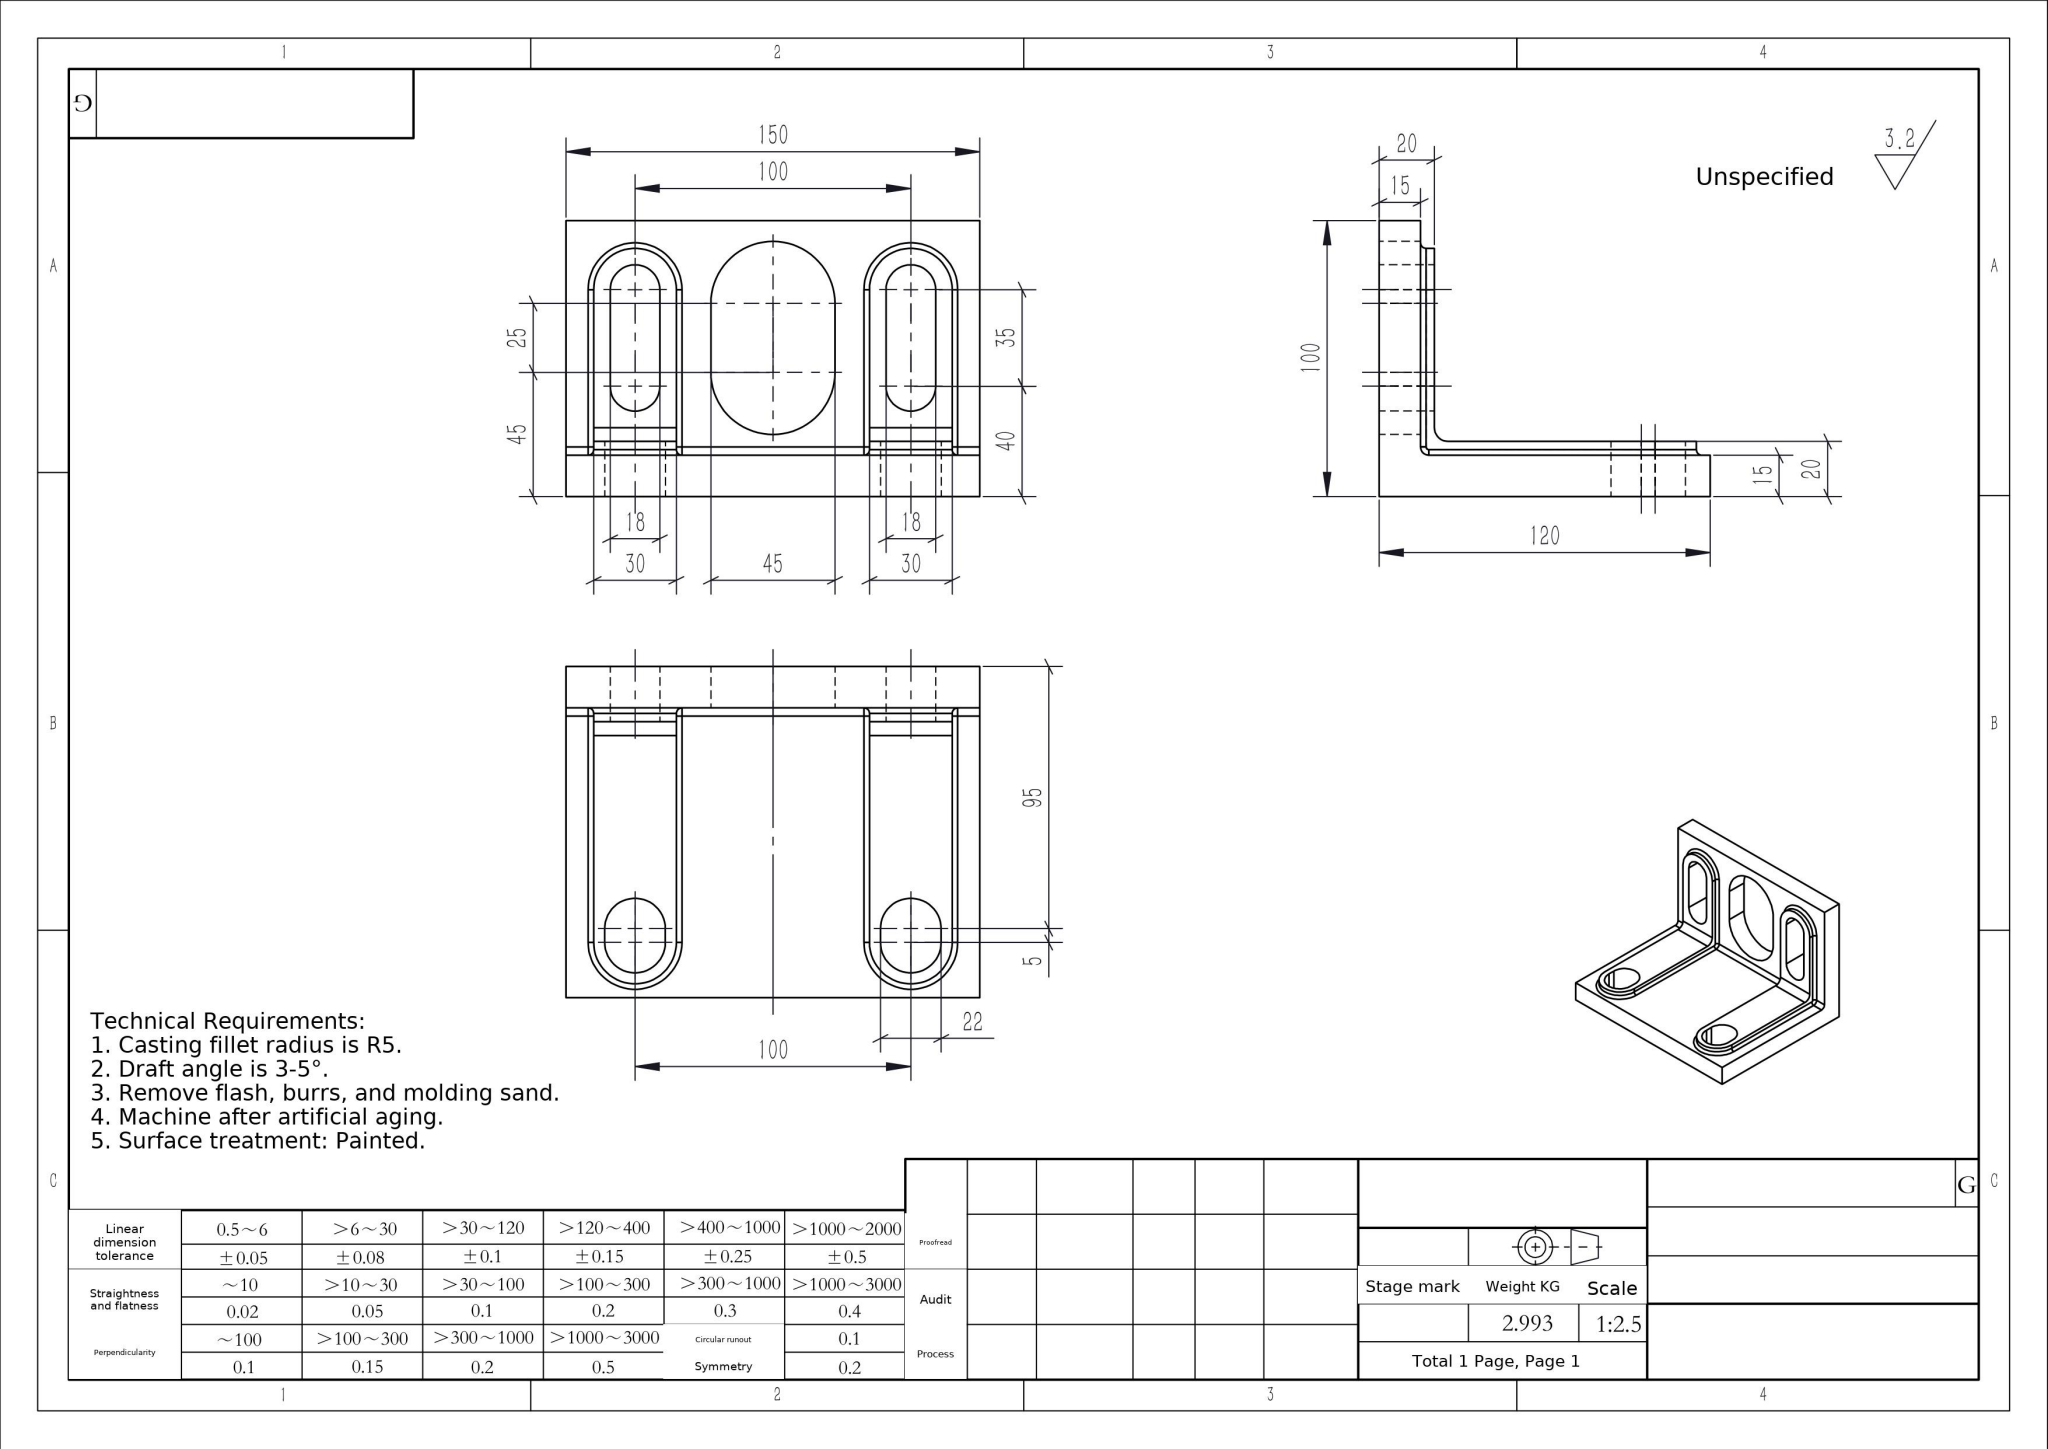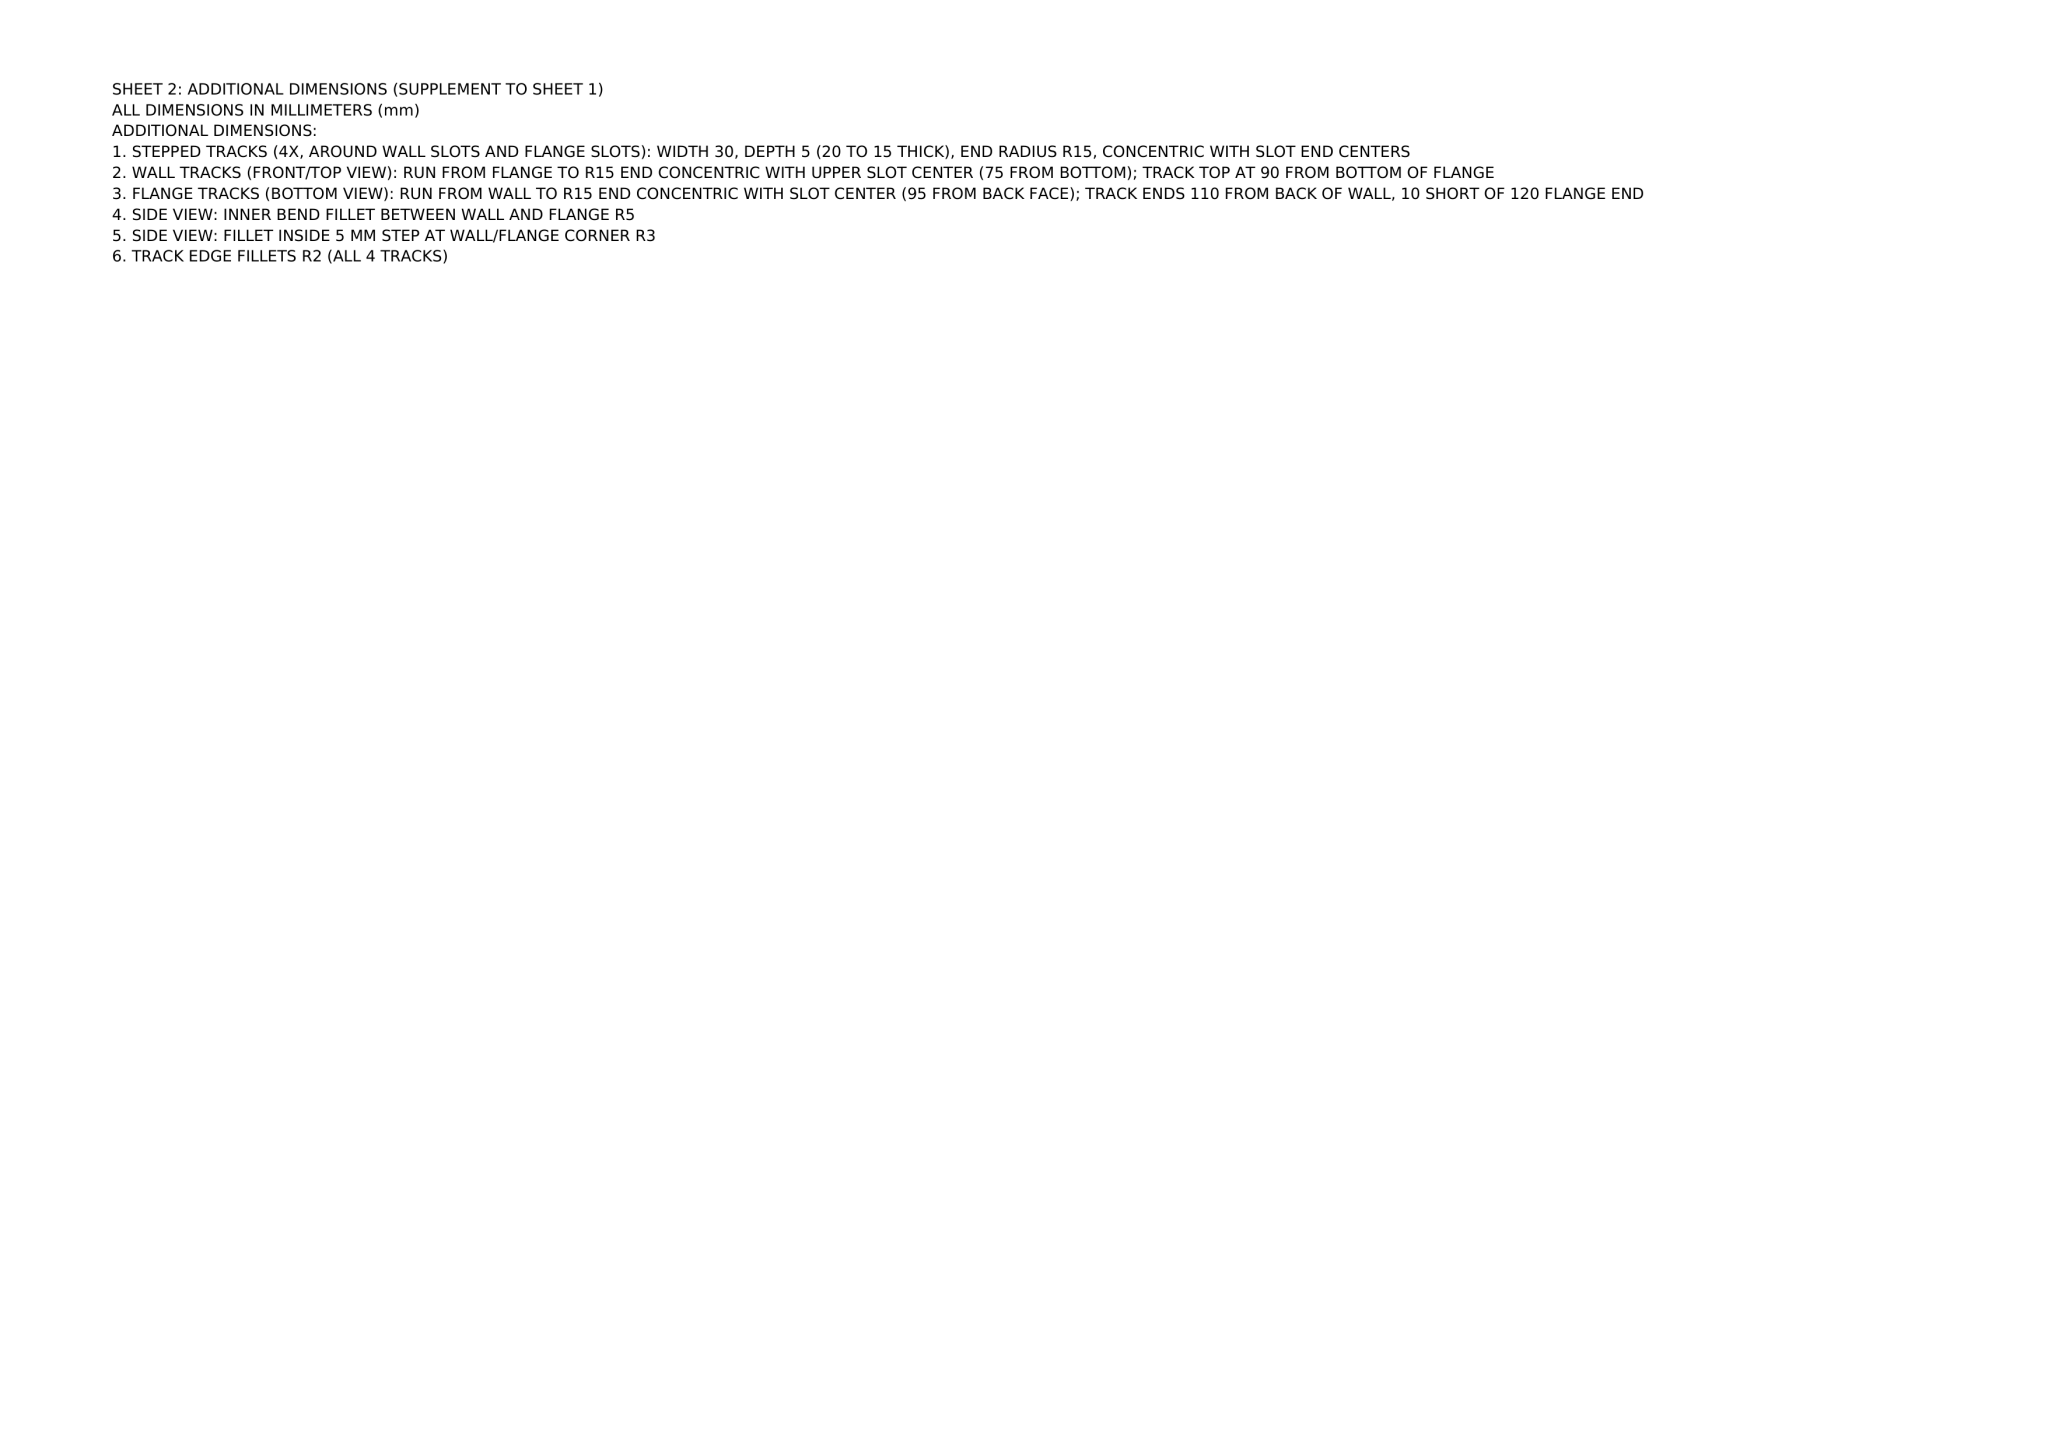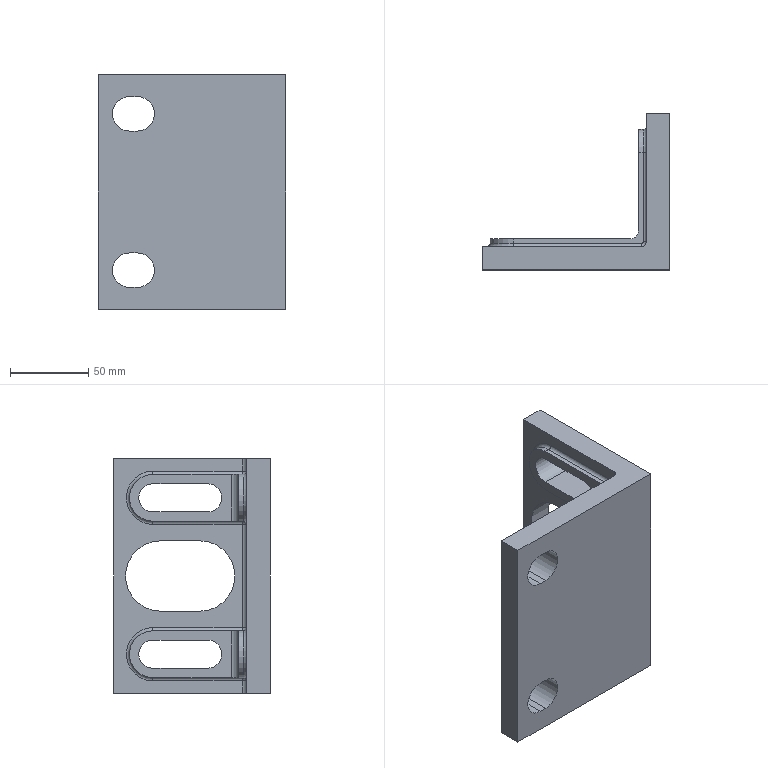Part | NX | mm | 1 solid | 61 faces | box 120 x 100 x 150 mm | volume 415756 mm3 | cylinder 27 | plane 26 | torus 8 | commonest cylinder face diameters 4 x8 30 x4 18 x4 22 x4 6 x3 45 x2 10 x2